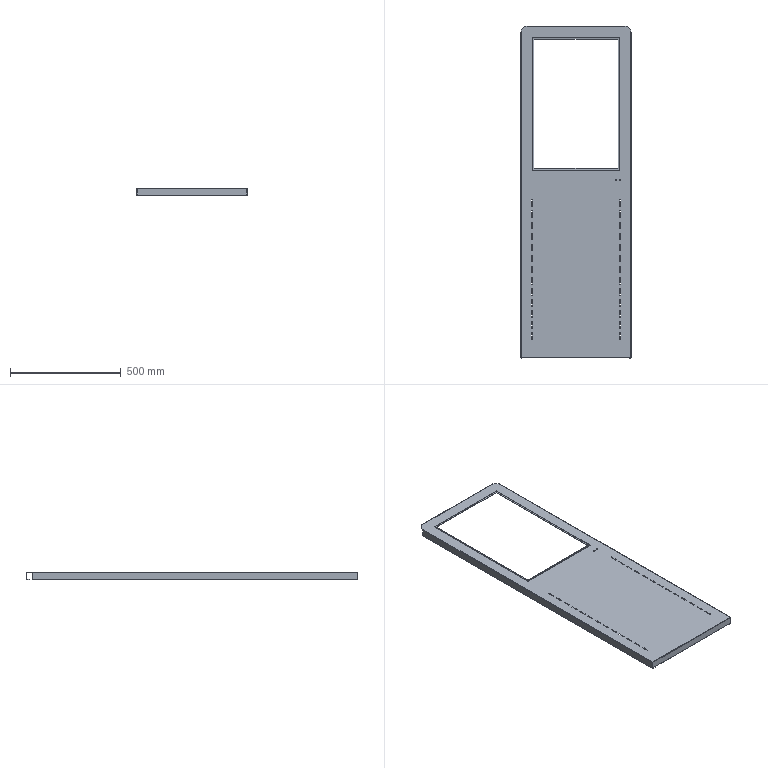Component | SolidWorks | w2-1 | 1 solid | 258 faces | volume 701071 mm3 | plane 210 | cylinder 40 | spline 8 | commonest cylinder face diameters 3 x11 1 x11 2.2 x6 0.2 x6 5 x4 57 x2